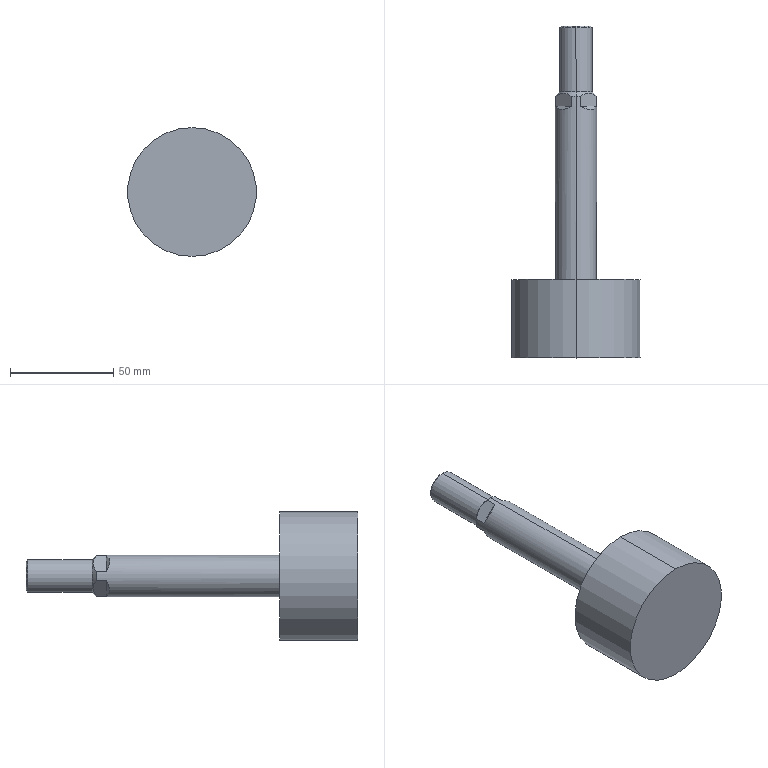Component | SolidWorks | NewCurveBenderSC63x40Cylinder-DoubleWheel-1_NewTypeCurveBenderSC-63x40(0)_r-DoubleWheel-1 | 1 solid | 21 faces | box 62.5 x 161 x 62.5 mm | volume 151202 mm3 | plane 11 | cylinder 6 | cone 4 | commonest cylinder face diameters 62.5 x2 20 x2 16 x2
build123d program:
from build123d import *

# Parameters (mm, degrees)
CUT_EXTRUDE1_DEPTH      = 17
CUT_EXTRUDE1_DEPTH_BACK = 17
CUT_EXTRUDE2_DEPTH      = 17
CUT_EXTRUDE2_DEPTH_BACK = 17


with BuildPart() as part:
    # Sketch1 → Revolve1 (revolve)
    with BuildSketch(Plane.XY, mode=Mode.PRIVATE) as revolve1_sk:
        Polygon((-57, 0), (-57, 7.08), (-56.08, 8), (-25, 8), (-23, 10), (66, 10), (66, 31.25), (104, 31.25), (104, 0), align=None)
    revolve(revolve1_sk.sketch.rotate(Axis((104, 0, 0), (-1, 0, 0)), 270), axis=Axis((104, 0, 0), (-1, 0, 0)))

    # Sketch2 → Cut-Extrude1 (cut, two sides: drawn at the far end of the back side and taken through both)
    with BuildSketch(Plane(origin=(0, 0, 0), x_dir=(1, 0, 0), z_dir=(0, -0.7071, 0.7071)).offset(-CUT_EXTRUDE1_DEPTH_BACK)):
        Polygon((-74, -25.5), (-1, -25.5), (-18, -8.5), (-57, -8.5), (-57, 8.5), (-18, 8.5), (-1, 25.5), (-74, 25.5), align=None)
    extrude(amount=CUT_EXTRUDE1_DEPTH + CUT_EXTRUDE1_DEPTH_BACK, mode=Mode.SUBTRACT)

    # Sketch3 → Cut-Extrude2 (cut, two sides: drawn at the far end of the back side and taken through both)
    with BuildSketch(Plane(origin=(0, 0, 0), x_dir=(-1, 0, 0), z_dir=(0, -0.7071, -0.7071)).offset(-CUT_EXTRUDE2_DEPTH_BACK)):
        Polygon((74, 25.5), (1, 25.5), (18, 8.5), (57, 8.5), (57, -8.5), (18, -8.5), (1, -25.5), (74, -25.5), align=None)
    extrude(amount=CUT_EXTRUDE2_DEPTH + CUT_EXTRUDE2_DEPTH_BACK, mode=Mode.SUBTRACT)


solid = part.part

# Placed as in the assembly
solid = solid.moved(Location((50, -301, 0), (0, 0, -90)))
STEP:
#1=CARTESIAN_POINT('',(1.969,-15.945,1.23));
#2=VERTEX_POINT('',#1);
#3=CARTESIAN_POINT('',(1.969,-15.945,-1.23));
#4=VERTEX_POINT('',#3);
#5=CARTESIAN_POINT('',(1.969,-15.945,0.));
#6=DIRECTION('',(-0.,1.,0.));
#7=DIRECTION('',(0.,0.,1.));
#8=AXIS2_PLACEMENT_3D('',#5,#6,#7);
#9=CIRCLE('',#8,1.23);
#10=EDGE_CURVE('',#2,#4,#9,.T.);
#11=ORIENTED_EDGE('',*,*,#10,.T.);
#12=CARTESIAN_POINT('',(1.969,-14.449,-1.23));
#13=VERTEX_POINT('',#12);
#14=CARTESIAN_POINT('',(1.969,-15.945,-1.23));
#15=DIRECTION('',(-0.,1.,0.));
#16=VECTOR('',#15,39.37);
#17=LINE('',#14,#16);
#18=EDGE_CURVE('',#4,#13,#17,.T.);
#19=ORIENTED_EDGE('',*,*,#18,.T.);
#20=CARTESIAN_POINT('',(1.969,-14.449,1.23));
#21=VERTEX_POINT('',#20);
#22=CARTESIAN_POINT('',(1.969,-14.449,0.));
#23=DIRECTION('',(-0.,1.,0.));
#24=DIRECTION('',(0.,0.,1.));
#25=AXIS2_PLACEMENT_3D('',#22,#23,#24);
#26=CIRCLE('',#25,1.23);
#27=EDGE_CURVE('',#21,#13,#26,.T.);
#28=ORIENTED_EDGE('',*,*,#27,.F.);
#29=CARTESIAN_POINT('',(1.969,-15.945,1.23));
#30=DIRECTION('',(-0.,1.,0.));
#31=VECTOR('',#30,39.37);
#32=LINE('',#29,#31);
#33=EDGE_CURVE('',#2,#21,#32,.T.);
#34=ORIENTED_EDGE('',*,*,#33,.F.);
#35=EDGE_LOOP('',(#11,#19,#28,#34));
#36=FACE_OUTER_BOUND('',#35,.T.);
#37=CARTESIAN_POINT('',(1.969,-15.945,0.));
#38=DIRECTION('',(-0.,1.,0.));
#39=DIRECTION('',(0.,0.,1.));
#40=AXIS2_PLACEMENT_3D('',#37,#38,#39);
#41=CYLINDRICAL_SURFACE('',#40,1.23);
#42=ADVANCED_FACE('',(#36),#41,.T.);
#43=CARTESIAN_POINT('',(1.969,-14.449,0.3937));
#44=VERTEX_POINT('',#43);
#45=CARTESIAN_POINT('',(1.969,-14.449,-0.3937));
#46=VERTEX_POINT('',#45);
#47=CARTESIAN_POINT('',(1.969,-14.449,0.));
#48=DIRECTION('',(-0.,1.,0.));
#49=DIRECTION('',(0.,0.,1.));
#50=AXIS2_PLACEMENT_3D('',#47,#48,#49);
#51=CIRCLE('',#50,0.3937);
#52=EDGE_CURVE('',#44,#46,#51,.T.);
#53=ORIENTED_EDGE('',*,*,#52,.T.);
#54=CARTESIAN_POINT('',(1.969,-10.945,-0.3937));
#55=VERTEX_POINT('',#54);
#56=CARTESIAN_POINT('',(1.969,-15.945,-0.3937));
#57=DIRECTION('',(-0.,1.,0.));
#58=VECTOR('',#57,39.37);
#59=LINE('',#56,#58);
#60=EDGE_CURVE('',#46,#55,#59,.T.);
#61=ORIENTED_EDGE('',*,*,#60,.T.);
#62=CARTESIAN_POINT('',(2.058,-10.945,-0.3833));
#63=VERTEX_POINT('',#62);
#64=CARTESIAN_POINT('',(1.969,-10.945,0.));
#65=DIRECTION('',(-0.,1.,0.));
#66=DIRECTION('',(0.,0.,1.));
#67=AXIS2_PLACEMENT_3D('',#64,#65,#66);
#68=CIRCLE('',#67,0.3937);
#69=EDGE_CURVE('',#63,#55,#68,.T.);
#70=ORIENTED_EDGE('',*,*,#69,.F.);
#71=CARTESIAN_POINT('',(2.058,-11.142,-0.3833));
#72=VERTEX_POINT('',#71);
#73=CARTESIAN_POINT('',(2.058,-15.945,-0.3833));
#74=DIRECTION('',(0.,-1.,-0.));
#75=VECTOR('',#74,39.37);
#76=LINE('',#73,#75);
#77=EDGE_CURVE('',#63,#72,#76,.T.);
#78=ORIENTED_EDGE('',*,*,#77,.T.);
#79=CARTESIAN_POINT('',(2.352,-11.142,-0.08998));
#80=VERTEX_POINT('',#79);
#81=CARTESIAN_POINT('',(2.058,-11.142,-0.3833));
#82=CARTESIAN_POINT('',(2.208,-11.223,-0.3482));
#83=CARTESIAN_POINT('',(2.317,-11.223,-0.2395));
#84=CARTESIAN_POINT('',(2.352,-11.142,-0.08998));
#85=(BOUNDED_CURVE()B_SPLINE_CURVE(3,(#81,#82,#83,#84),.UNSPECIFIED.,.F.,.F.)B_SPLINE_CURVE_WITH_KNOTS((4,4),(2.587,3.696),.UNSPECIFIED.)CURVE()GEOMETRIC_REPRESENTATION_ITEM()RATIONAL_B_SPLINE_CURVE((1.,0.9,0.9,1.))REPRESENTATION_ITEM(''));
#86=EDGE_CURVE('',#72,#80,#85,.T.);
#87=ORIENTED_EDGE('',*,*,#86,.T.);
#88=CARTESIAN_POINT('',(2.352,-10.945,-0.08998));
#89=VERTEX_POINT('',#88);
#90=CARTESIAN_POINT('',(2.352,-15.945,-0.08998));
#91=DIRECTION('',(-0.,1.,0.));
#92=VECTOR('',#91,39.37);
#93=LINE('',#90,#92);
#94=EDGE_CURVE('',#80,#89,#93,.T.);
#95=ORIENTED_EDGE('',*,*,#94,.T.);
#96=CARTESIAN_POINT('',(2.352,-10.945,0.08998));
#97=VERTEX_POINT('',#96);
#98=CARTESIAN_POINT('',(1.969,-10.945,0.));
#99=DIRECTION('',(-0.,1.,0.));
#100=DIRECTION('',(0.,0.,1.));
#101=AXIS2_PLACEMENT_3D('',#98,#99,#100);
#102=CIRCLE('',#101,0.3937);
#103=EDGE_CURVE('',#97,#89,#102,.T.);
#104=ORIENTED_EDGE('',*,*,#103,.F.);
#105=CARTESIAN_POINT('',(2.352,-11.142,0.08998));
#106=VERTEX_POINT('',#105);
#107=CARTESIAN_POINT('',(2.352,-15.945,0.08998));
#108=DIRECTION('',(0.,-1.,-0.));
#109=VECTOR('',#108,39.37);
#110=LINE('',#107,#109);
#111=EDGE_CURVE('',#97,#106,#110,.T.);
#112=ORIENTED_EDGE('',*,*,#111,.T.);
#113=CARTESIAN_POINT('',(2.058,-11.142,0.3833));
#114=VERTEX_POINT('',#113);
#115=CARTESIAN_POINT('',(2.352,-11.142,0.08998));
#116=CARTESIAN_POINT('',(2.317,-11.223,0.2395));
#117=CARTESIAN_POINT('',(2.208,-11.223,0.3482));
#118=CARTESIAN_POINT('',(2.058,-11.142,0.3833));
#119=(BOUNDED_CURVE()B_SPLINE_CURVE(3,(#115,#116,#117,#118),.UNSPECIFIED.,.F.,.F.)B_SPLINE_CURVE_WITH_KNOTS((4,4),(2.587,3.696),.UNSPECIFIED.)CURVE()GEOMETRIC_REPRESENTATION_ITEM()RATIONAL_B_SPLINE_CURVE((1.,0.9,0.9,1.))REPRESENTATION_ITEM(''));
#120=EDGE_CURVE('',#106,#114,#119,.T.);
#121=ORIENTED_EDGE('',*,*,#120,.T.);
#122=CARTESIAN_POINT('',(2.058,-10.945,0.3833));
#123=VERTEX_POINT('',#122);
#124=CARTESIAN_POINT('',(2.058,-15.945,0.3833));
#125=DIRECTION('',(-0.,1.,0.));
#126=VECTOR('',#125,39.37);
#127=LINE('',#124,#126);
#128=EDGE_CURVE('',#114,#123,#127,.T.);
#129=ORIENTED_EDGE('',*,*,#128,.T.);
#130=CARTESIAN_POINT('',(1.969,-10.945,0.3937));
#131=VERTEX_POINT('',#130);
#132=CARTESIAN_POINT('',(1.969,-10.945,0.));
#133=DIRECTION('',(-0.,1.,0.));
#134=DIRECTION('',(0.,0.,1.));
#135=AXIS2_PLACEMENT_3D('',#132,#133,#134);
#136=CIRCLE('',#135,0.3937);
#137=EDGE_CURVE('',#131,#123,#136,.T.);
#138=ORIENTED_EDGE('',*,*,#137,.F.);
#139=CARTESIAN_POINT('',(1.969,-15.945,0.3937));
#140=DIRECTION('',(-0.,1.,0.));
#141=VECTOR('',#140,39.37);
#142=LINE('',#139,#141);
#143=EDGE_CURVE('',#44,#131,#142,.T.);
#144=ORIENTED_EDGE('',*,*,#143,.F.);
#145=EDGE_LOOP('',(#53,#61,#70,#78,#87,#95,#104,#112,#121,#129,#138,#144));
#146=FACE_OUTER_BOUND('',#145,.T.);
#147=CARTESIAN_POINT('',(1.969,-15.945,0.));
#148=DIRECTION('',(-0.,1.,0.));
#149=DIRECTION('',(0.,0.,1.));
#150=AXIS2_PLACEMENT_3D('',#147,#148,#149);
#151=CYLINDRICAL_SURFACE('',#150,0.3937);
#152=ADVANCED_FACE('',(#146),#151,.T.);
#153=CARTESIAN_POINT('',(1.969,-10.866,0.315));
#154=VERTEX_POINT('',#153);
#155=CARTESIAN_POINT('',(1.969,-10.866,-0.315));
#156=VERTEX_POINT('',#155);
#157=CARTESIAN_POINT('',(1.969,-10.866,0.));
#158=DIRECTION('',(-0.,1.,0.));
#159=DIRECTION('',(0.,0.,1.));
#160=AXIS2_PLACEMENT_3D('',#157,#158,#159);
#161=CIRCLE('',#160,0.315);
#162=EDGE_CURVE('',#154,#156,#161,.T.);
#163=ORIENTED_EDGE('',*,*,#162,.F.);
#164=CARTESIAN_POINT('',(1.969,-10.945,0.3937));
#165=DIRECTION('',(0.,-0.7071,0.7071));
#166=VECTOR('',#165,39.37);
#167=LINE('',#164,#166);
#168=EDGE_CURVE('',#154,#131,#167,.T.);
#169=ORIENTED_EDGE('',*,*,#168,.T.);
#170=ORIENTED_EDGE('',*,*,#137,.T.);
#171=CARTESIAN_POINT('',(2.058,-10.945,0.3833));
#172=CARTESIAN_POINT('',(2.081,-10.928,0.3605));
#173=CARTESIAN_POINT('',(2.105,-10.913,0.337));
#174=CARTESIAN_POINT('',(2.141,-10.897,0.3003));
#175=CARTESIAN_POINT('',(2.154,-10.893,0.2878));
#176=CARTESIAN_POINT('',(2.18,-10.887,0.2622));
#177=CARTESIAN_POINT('',(2.192,-10.886,0.2494));
#178=CARTESIAN_POINT('',(2.218,-10.886,0.2239));
#179=CARTESIAN_POINT('',(2.231,-10.887,0.2111));
#180=CARTESIAN_POINT('',(2.256,-10.893,0.1855));
#181=CARTESIAN_POINT('',(2.269,-10.897,0.173));
#182=CARTESIAN_POINT('',(2.306,-10.913,0.1362));
#183=CARTESIAN_POINT('',(2.329,-10.928,0.1128));
#184=CARTESIAN_POINT('',(2.352,-10.945,0.08998));
#185=B_SPLINE_CURVE_WITH_KNOTS('',3,(#171,#172,#173,#174,#175,#176,#177,#178,#179,#180,#181,#182,#183,#184),.UNSPECIFIED.,.F.,.F.,(4,2,2,2,2,2,4),(0.00000043,0.002754,0.004131,0.005507,0.006884,0.008261,0.01101),.UNSPECIFIED.);
#186=EDGE_CURVE('',#123,#97,#185,.T.);
#187=ORIENTED_EDGE('',*,*,#186,.T.);
#188=ORIENTED_EDGE('',*,*,#103,.T.);
#189=CARTESIAN_POINT('',(2.352,-10.945,-0.08998));
#190=CARTESIAN_POINT('',(2.329,-10.928,-0.1128));
#191=CARTESIAN_POINT('',(2.306,-10.913,-0.1362));
#192=CARTESIAN_POINT('',(2.269,-10.897,-0.1729));
#193=CARTESIAN_POINT('',(2.256,-10.893,-0.1855));
#194=CARTESIAN_POINT('',(2.231,-10.887,-0.211));
#195=CARTESIAN_POINT('',(2.218,-10.886,-0.2238));
#196=CARTESIAN_POINT('',(2.192,-10.886,-0.2494));
#197=CARTESIAN_POINT('',(2.18,-10.887,-0.2622));
#198=CARTESIAN_POINT('',(2.154,-10.893,-0.2877));
#199=CARTESIAN_POINT('',(2.141,-10.897,-0.3003));
#200=CARTESIAN_POINT('',(2.105,-10.913,-0.337));
#201=CARTESIAN_POINT('',(2.081,-10.928,-0.3605));
#202=CARTESIAN_POINT('',(2.058,-10.945,-0.3833));
#203=B_SPLINE_CURVE_WITH_KNOTS('',3,(#189,#190,#191,#192,#193,#194,#195,#196,#197,#198,#199,#200,#201,#202),.UNSPECIFIED.,.F.,.F.,(4,2,2,2,2,2,4),(0.00000043,0.002754,0.004131,0.005507,0.006884,0.008261,0.01101),.UNSPECIFIED.);
#204=EDGE_CURVE('',#89,#63,#203,.T.);
#205=ORIENTED_EDGE('',*,*,#204,.T.);
#206=ORIENTED_EDGE('',*,*,#69,.T.);
#207=CARTESIAN_POINT('',(1.969,-10.945,-0.3937));
#208=DIRECTION('',(0.,-0.7071,-0.7071));
#209=VECTOR('',#208,39.37);
#210=LINE('',#207,#209);
#211=EDGE_CURVE('',#156,#55,#210,.T.);
#212=ORIENTED_EDGE('',*,*,#211,.F.);
#213=EDGE_LOOP('',(#163,#169,#170,#187,#188,#205,#206,#212));
#214=FACE_OUTER_BOUND('',#213,.T.);
#215=CARTESIAN_POINT('',(1.969,-10.945,0.));
#216=DIRECTION('',(0.,-1.,-0.));
#217=DIRECTION('',(0.,0.,-1.));
#218=AXIS2_PLACEMENT_3D('',#215,#216,#217);
#219=CONICAL_SURFACE('',#218,0.3937,0.7854);
#220=ADVANCED_FACE('',(#214),#219,.T.);
#221=ORIENTED_EDGE('',*,*,#162,.T.);
#222=CARTESIAN_POINT('',(1.969,-9.643,-0.315));
#223=VERTEX_POINT('',#222);
#224=CARTESIAN_POINT('',(1.969,-15.945,-0.315));
#225=DIRECTION('',(-0.,1.,0.));
#226=VECTOR('',#225,39.37);
#227=LINE('',#224,#226);
#228=EDGE_CURVE('',#156,#223,#227,.T.);
#229=ORIENTED_EDGE('',*,*,#228,.T.);
#230=CARTESIAN_POINT('',(1.969,-9.643,0.315));
#231=VERTEX_POINT('',#230);
#232=CARTESIAN_POINT('',(1.969,-9.643,0.));
#233=DIRECTION('',(-0.,1.,0.));
#234=DIRECTION('',(0.,0.,1.));
#235=AXIS2_PLACEMENT_3D('',#232,#233,#234);
#236=CIRCLE('',#235,0.315);
#237=EDGE_CURVE('',#231,#223,#236,.T.);
#238=ORIENTED_EDGE('',*,*,#237,.F.);
#239=CARTESIAN_POINT('',(1.969,-15.945,0.315));
#240=DIRECTION('',(-0.,1.,0.));
#241=VECTOR('',#240,39.37);
#242=LINE('',#239,#241);
#243=EDGE_CURVE('',#154,#231,#242,.T.);
#244=ORIENTED_EDGE('',*,*,#243,.F.);
#245=EDGE_LOOP('',(#221,#229,#238,#244));
#246=FACE_OUTER_BOUND('',#245,.T.);
#247=CARTESIAN_POINT('',(1.969,-15.945,0.));
#248=DIRECTION('',(-0.,1.,0.));
#249=DIRECTION('',(0.,0.,1.));
#250=AXIS2_PLACEMENT_3D('',#247,#248,#249);
#251=CYLINDRICAL_SURFACE('',#250,0.315);
#252=ADVANCED_FACE('',(#246),#251,.T.);
#253=CARTESIAN_POINT('',(1.969,-9.606,0.2787));
#254=VERTEX_POINT('',#253);
#255=CARTESIAN_POINT('',(1.969,-9.606,-0.2787));
#256=VERTEX_POINT('',#255);
#257=CARTESIAN_POINT('',(1.969,-9.606,0.));
#258=DIRECTION('',(-0.,1.,0.));
#259=DIRECTION('',(0.,0.,1.));
#260=AXIS2_PLACEMENT_3D('',#257,#258,#259);
#261=CIRCLE('',#260,0.2787);
#262=EDGE_CURVE('',#254,#256,#261,.T.);
#263=ORIENTED_EDGE('',*,*,#262,.F.);
#264=CARTESIAN_POINT('',(1.969,-9.643,0.315));
#265=DIRECTION('',(0.,-0.7071,0.7071));
#266=VECTOR('',#265,39.37);
#267=LINE('',#264,#266);
#268=EDGE_CURVE('',#254,#231,#267,.T.);
#269=ORIENTED_EDGE('',*,*,#268,.T.);
#270=ORIENTED_EDGE('',*,*,#237,.T.);
#271=CARTESIAN_POINT('',(1.969,-9.643,-0.315));
#272=DIRECTION('',(0.,-0.7071,-0.7071));
#273=VECTOR('',#272,39.37);
#274=LINE('',#271,#273);
#275=EDGE_CURVE('',#256,#223,#274,.T.);
#276=ORIENTED_EDGE('',*,*,#275,.F.);
#277=EDGE_LOOP('',(#263,#269,#270,#276));
#278=FACE_OUTER_BOUND('',#277,.T.);
#279=CARTESIAN_POINT('',(1.969,-9.643,0.));
#280=DIRECTION('',(0.,-1.,-0.));
#281=DIRECTION('',(0.,0.,-1.));
#282=AXIS2_PLACEMENT_3D('',#279,#280,#281);
#283=CONICAL_SURFACE('',#282,0.315,0.7854);
#284=ADVANCED_FACE('',(#278),#283,.T.);
#285=CARTESIAN_POINT('',(1.969,-9.606,0.));
#286=DIRECTION('',(-0.,1.,0.));
#287=DIRECTION('',(0.,0.,1.));
#288=AXIS2_PLACEMENT_3D('',#285,#286,#287);
#289=CIRCLE('',#288,0.2787);
#290=EDGE_CURVE('',#256,#254,#289,.T.);
#291=ORIENTED_EDGE('',*,*,#290,.T.);
#292=ORIENTED_EDGE('',*,*,#262,.T.);
#293=EDGE_LOOP('',(#291,#292));
#294=FACE_OUTER_BOUND('',#293,.T.);
#295=CARTESIAN_POINT('',(1.969,-9.606,0.));
#296=DIRECTION('',(0.,-1.,0.));
#297=DIRECTION('',(0.,-0.,-1.));
#298=AXIS2_PLACEMENT_3D('',#295,#296,#297);
#299=PLANE('',#298);
#300=ADVANCED_FACE('',(#294),#299,.F.);
#301=ORIENTED_EDGE('',*,*,#268,.F.);
#302=ORIENTED_EDGE('',*,*,#290,.F.);
#303=ORIENTED_EDGE('',*,*,#275,.T.);
#304=CARTESIAN_POINT('',(1.969,-9.643,0.));
#305=DIRECTION('',(-0.,1.,0.));
#306=DIRECTION('',(0.,0.,1.));
#307=AXIS2_PLACEMENT_3D('',#304,#305,#306);
#308=CIRCLE('',#307,0.315);
#309=EDGE_CURVE('',#223,#231,#308,.T.);
#310=ORIENTED_EDGE('',*,*,#309,.T.);
#311=EDGE_LOOP('',(#301,#302,#303,#310));
#312=FACE_OUTER_BOUND('',#311,.T.);
#313=CARTESIAN_POINT('',(1.969,-9.643,0.));
#314=DIRECTION('',(0.,-1.,-0.));
#315=DIRECTION('',(0.,0.,-1.));
#316=AXIS2_PLACEMENT_3D('',#313,#314,#315);
#317=CONICAL_SURFACE('',#316,0.315,0.7854);
#318=ADVANCED_FACE('',(#312),#317,.T.);
#319=ORIENTED_EDGE('',*,*,#228,.F.);
#320=CARTESIAN_POINT('',(1.969,-10.866,0.));
#321=DIRECTION('',(-0.,1.,0.));
#322=DIRECTION('',(0.,0.,1.));
#323=AXIS2_PLACEMENT_3D('',#320,#321,#322);
#324=CIRCLE('',#323,0.315);
#325=EDGE_CURVE('',#156,#154,#324,.T.);
#326=ORIENTED_EDGE('',*,*,#325,.T.);
#327=ORIENTED_EDGE('',*,*,#243,.T.);
#328=ORIENTED_EDGE('',*,*,#309,.F.);
#329=EDGE_LOOP('',(#319,#326,#327,#328));
#330=FACE_OUTER_BOUND('',#329,.T.);
#331=CARTESIAN_POINT('',(1.969,-15.945,0.));
#332=DIRECTION('',(-0.,1.,0.));
#333=DIRECTION('',(0.,0.,1.));
#334=AXIS2_PLACEMENT_3D('',#331,#332,#333);
#335=CYLINDRICAL_SURFACE('',#334,0.315);
#336=ADVANCED_FACE('',(#330),#335,.T.);
#337=ORIENTED_EDGE('',*,*,#168,.F.);
#338=ORIENTED_EDGE('',*,*,#325,.F.);
#339=ORIENTED_EDGE('',*,*,#211,.T.);
#340=CARTESIAN_POINT('',(1.879,-10.945,-0.3833));
#341=VERTEX_POINT('',#340);
#342=CARTESIAN_POINT('',(1.969,-10.945,0.));
#343=DIRECTION('',(-0.,1.,0.));
#344=DIRECTION('',(0.,0.,1.));
#345=AXIS2_PLACEMENT_3D('',#342,#343,#344);
#346=CIRCLE('',#345,0.3937);
#347=EDGE_CURVE('',#55,#341,#346,.T.);
#348=ORIENTED_EDGE('',*,*,#347,.T.);
#349=CARTESIAN_POINT('',(1.585,-10.945,-0.08998));
#350=VERTEX_POINT('',#349);
#351=CARTESIAN_POINT('',(1.879,-10.945,-0.3833));
#352=CARTESIAN_POINT('',(1.856,-10.928,-0.3605));
#353=CARTESIAN_POINT('',(1.832,-10.913,-0.337));
#354=CARTESIAN_POINT('',(1.796,-10.897,-0.3003));
#355=CARTESIAN_POINT('',(1.783,-10.893,-0.2878));
#356=CARTESIAN_POINT('',(1.757,-10.887,-0.2622));
#357=CARTESIAN_POINT('',(1.745,-10.886,-0.2494));
#358=CARTESIAN_POINT('',(1.719,-10.886,-0.2239));
#359=CARTESIAN_POINT('',(1.706,-10.887,-0.2111));
#360=CARTESIAN_POINT('',(1.681,-10.893,-0.1855));
#361=CARTESIAN_POINT('',(1.668,-10.897,-0.173));
#362=CARTESIAN_POINT('',(1.631,-10.913,-0.1362));
#363=CARTESIAN_POINT('',(1.608,-10.928,-0.1128));
#364=CARTESIAN_POINT('',(1.585,-10.945,-0.08998));
#365=B_SPLINE_CURVE_WITH_KNOTS('',3,(#351,#352,#353,#354,#355,#356,#357,#358,#359,#360,#361,#362,#363,#364),.UNSPECIFIED.,.F.,.F.,(4,2,2,2,2,2,4),(0.00000043,0.002754,0.004131,0.005507,0.006884,0.008261,0.01101),.UNSPECIFIED.);
#366=EDGE_CURVE('',#341,#350,#365,.T.);
#367=ORIENTED_EDGE('',*,*,#366,.T.);
#368=CARTESIAN_POINT('',(1.585,-10.945,0.08998));
#369=VERTEX_POINT('',#368);
#370=CARTESIAN_POINT('',(1.969,-10.945,0.));
#371=DIRECTION('',(-0.,1.,0.));
#372=DIRECTION('',(0.,0.,1.));
#373=AXIS2_PLACEMENT_3D('',#370,#371,#372);
#374=CIRCLE('',#373,0.3937);
#375=EDGE_CURVE('',#350,#369,#374,.T.);
#376=ORIENTED_EDGE('',*,*,#375,.T.);
#377=CARTESIAN_POINT('',(1.879,-10.945,0.3833));
#378=VERTEX_POINT('',#377);
#379=CARTESIAN_POINT('',(1.585,-10.945,0.08998));
#380=CARTESIAN_POINT('',(1.608,-10.928,0.1128));
#381=CARTESIAN_POINT('',(1.631,-10.913,0.1362));
#382=CARTESIAN_POINT('',(1.668,-10.897,0.1729));
#383=CARTESIAN_POINT('',(1.681,-10.893,0.1855));
#384=CARTESIAN_POINT('',(1.706,-10.887,0.211));
#385=CARTESIAN_POINT('',(1.719,-10.886,0.2238));
#386=CARTESIAN_POINT('',(1.745,-10.886,0.2494));
#387=CARTESIAN_POINT('',(1.757,-10.887,0.2622));
#388=CARTESIAN_POINT('',(1.783,-10.893,0.2877));
#389=CARTESIAN_POINT('',(1.796,-10.897,0.3003));
#390=CARTESIAN_POINT('',(1.832,-10.913,0.337));
#391=CARTESIAN_POINT('',(1.856,-10.928,0.3605));
#392=CARTESIAN_POINT('',(1.879,-10.945,0.3833));
#393=B_SPLINE_CURVE_WITH_KNOTS('',3,(#379,#380,#381,#382,#383,#384,#385,#386,#387,#388,#389,#390,#391,#392),.UNSPECIFIED.,.F.,.F.,(4,2,2,2,2,2,4),(0.00000043,0.002754,0.004131,0.005507,0.006884,0.008261,0.01101),.UNSPECIFIED.);
#394=EDGE_CURVE('',#369,#378,#393,.T.);
#395=ORIENTED_EDGE('',*,*,#394,.T.);
#396=CARTESIAN_POINT('',(1.969,-10.945,0.));
#397=DIRECTION('',(-0.,1.,0.));
#398=DIRECTION('',(0.,0.,1.));
#399=AXIS2_PLACEMENT_3D('',#396,#397,#398);
#400=CIRCLE('',#399,0.3937);
#401=EDGE_CURVE('',#378,#131,#400,.T.);
#402=ORIENTED_EDGE('',*,*,#401,.T.);
#403=EDGE_LOOP('',(#337,#338,#339,#348,#367,#376,#395,#402));
#404=FACE_OUTER_BOUND('',#403,.T.);
#405=CARTESIAN_POINT('',(1.969,-10.945,0.));
#406=DIRECTION('',(0.,-1.,-0.));
#407=DIRECTION('',(0.,0.,-1.));
#408=AXIS2_PLACEMENT_3D('',#405,#406,#407);
#409=CONICAL_SURFACE('',#408,0.3937,0.7854);
#410=ADVANCED_FACE('',(#404),#409,.T.);
#411=ORIENTED_EDGE('',*,*,#60,.F.);
#412=CARTESIAN_POINT('',(1.969,-14.449,0.));
#413=DIRECTION('',(-0.,1.,0.));
#414=DIRECTION('',(0.,0.,1.));
#415=AXIS2_PLACEMENT_3D('',#412,#413,#414);
#416=CIRCLE('',#415,0.3937);
#417=EDGE_CURVE('',#46,#44,#416,.T.);
#418=ORIENTED_EDGE('',*,*,#417,.T.);
#419=ORIENTED_EDGE('',*,*,#143,.T.);
#420=ORIENTED_EDGE('',*,*,#401,.F.);
#421=CARTESIAN_POINT('',(1.879,-11.142,0.3833));
#422=VERTEX_POINT('',#421);
#423=CARTESIAN_POINT('',(1.879,-15.945,0.3833));
#424=DIRECTION('',(0.,-1.,-0.));
#425=VECTOR('',#424,39.37);
#426=LINE('',#423,#425);
#427=EDGE_CURVE('',#378,#422,#426,.T.);
#428=ORIENTED_EDGE('',*,*,#427,.T.);
#429=CARTESIAN_POINT('',(1.585,-11.142,0.08998));
#430=VERTEX_POINT('',#429);
#431=CARTESIAN_POINT('',(1.879,-11.142,0.3833));
#432=CARTESIAN_POINT('',(1.729,-11.223,0.3482));
#433=CARTESIAN_POINT('',(1.62,-11.223,0.2395));
#434=CARTESIAN_POINT('',(1.585,-11.142,0.08998));
#435=(BOUNDED_CURVE()B_SPLINE_CURVE(3,(#431,#432,#433,#434),.UNSPECIFIED.,.F.,.F.)B_SPLINE_CURVE_WITH_KNOTS((4,4),(2.587,3.696),.UNSPECIFIED.)CURVE()GEOMETRIC_REPRESENTATION_ITEM()RATIONAL_B_SPLINE_CURVE((1.,0.9,0.9,1.))REPRESENTATION_ITEM(''));
#436=EDGE_CURVE('',#422,#430,#435,.T.);
#437=ORIENTED_EDGE('',*,*,#436,.T.);
#438=CARTESIAN_POINT('',(1.585,-15.945,0.08998));
#439=DIRECTION('',(-0.,1.,0.));
#440=VECTOR('',#439,39.37);
#441=LINE('',#438,#440);
#442=EDGE_CURVE('',#430,#369,#441,.T.);
#443=ORIENTED_EDGE('',*,*,#442,.T.);
#444=ORIENTED_EDGE('',*,*,#375,.F.);
#445=CARTESIAN_POINT('',(1.585,-11.142,-0.08998));
#446=VERTEX_POINT('',#445);
#447=CARTESIAN_POINT('',(1.585,-15.945,-0.08998));
#448=DIRECTION('',(0.,-1.,-0.));
#449=VECTOR('',#448,39.37);
#450=LINE('',#447,#449);
#451=EDGE_CURVE('',#350,#446,#450,.T.);
#452=ORIENTED_EDGE('',*,*,#451,.T.);
#453=CARTESIAN_POINT('',(1.879,-11.142,-0.3833));
#454=VERTEX_POINT('',#453);
#455=CARTESIAN_POINT('',(1.585,-11.142,-0.08998));
#456=CARTESIAN_POINT('',(1.62,-11.223,-0.2395));
#457=CARTESIAN_POINT('',(1.729,-11.223,-0.3482));
#458=CARTESIAN_POINT('',(1.879,-11.142,-0.3833));
#459=(BOUNDED_CURVE()B_SPLINE_CURVE(3,(#455,#456,#457,#458),.UNSPECIFIED.,.F.,.T.)B_SPLINE_CURVE_WITH_KNOTS((4,4),(2.587,3.696),.UNSPECIFIED.)CURVE()GEOMETRIC_REPRESENTATION_ITEM()RATIONAL_B_SPLINE_CURVE((1.,0.9,0.9,1.))REPRESENTATION_ITEM(''));
#460=EDGE_CURVE('',#446,#454,#459,.T.);
#461=ORIENTED_EDGE('',*,*,#460,.T.);
#462=CARTESIAN_POINT('',(1.879,-15.945,-0.3833));
#463=DIRECTION('',(-0.,1.,0.));
#464=VECTOR('',#463,39.37);
#465=LINE('',#462,#464);
#466=EDGE_CURVE('',#454,#341,#465,.T.);
#467=ORIENTED_EDGE('',*,*,#466,.T.);
#468=ORIENTED_EDGE('',*,*,#347,.F.);
#469=EDGE_LOOP('',(#411,#418,#419,#420,#428,#437,#443,#444,#452,#461,#467,#468));
#470=FACE_OUTER_BOUND('',#469,.T.);
#471=CARTESIAN_POINT('',(1.969,-15.945,0.));
#472=DIRECTION('',(-0.,1.,0.));
#473=DIRECTION('',(0.,0.,1.));
#474=AXIS2_PLACEMENT_3D('',#471,#472,#473);
#475=CYLINDRICAL_SURFACE('',#474,0.3937);
#476=ADVANCED_FACE('',(#470),#475,.T.);
#477=ORIENTED_EDGE('',*,*,#52,.F.);
#478=ORIENTED_EDGE('',*,*,#417,.F.);
#479=EDGE_LOOP('',(#477,#478));
#480=FACE_BOUND('',#479,.T.);
#481=ORIENTED_EDGE('',*,*,#27,.T.);
#482=CARTESIAN_POINT('',(1.969,-14.449,0.));
#483=DIRECTION('',(-0.,1.,0.));
#484=DIRECTION('',(0.,0.,1.));
#485=AXIS2_PLACEMENT_3D('',#482,#483,#484);
#486=CIRCLE('',#485,1.23);
#487=EDGE_CURVE('',#13,#21,#486,.T.);
#488=ORIENTED_EDGE('',*,*,#487,.T.);
#489=EDGE_LOOP('',(#481,#488));
#490=FACE_OUTER_BOUND('',#489,.T.);
#491=CARTESIAN_POINT('',(2.362,-14.449,0.));
#492=DIRECTION('',(0.,-1.,0.));
#493=DIRECTION('',(0.,-0.,-1.));
#494=AXIS2_PLACEMENT_3D('',#491,#492,#493);
#495=PLANE('',#494);
#496=ADVANCED_FACE('',(#480,#490),#495,.F.);
#497=ORIENTED_EDGE('',*,*,#18,.F.);
#498=CARTESIAN_POINT('',(1.969,-15.945,0.));
#499=DIRECTION('',(-0.,1.,0.));
#500=DIRECTION('',(0.,0.,1.));
#501=AXIS2_PLACEMENT_3D('',#498,#499,#500);
#502=CIRCLE('',#501,1.23);
#503=EDGE_CURVE('',#4,#2,#502,.T.);
#504=ORIENTED_EDGE('',*,*,#503,.T.);
#505=ORIENTED_EDGE('',*,*,#33,.T.);
#506=ORIENTED_EDGE('',*,*,#487,.F.);
#507=EDGE_LOOP('',(#497,#504,#505,#506));
#508=FACE_OUTER_BOUND('',#507,.T.);
#509=CARTESIAN_POINT('',(1.969,-15.945,0.));
#510=DIRECTION('',(-0.,1.,0.));
#511=DIRECTION('',(0.,0.,1.));
#512=AXIS2_PLACEMENT_3D('',#509,#510,#511);
#513=CYLINDRICAL_SURFACE('',#512,1.23);
#514=ADVANCED_FACE('',(#508),#513,.T.);
#515=ORIENTED_EDGE('',*,*,#10,.F.);
#516=ORIENTED_EDGE('',*,*,#503,.F.);
#517=EDGE_LOOP('',(#515,#516));
#518=FACE_OUTER_BOUND('',#517,.T.);
#519=CARTESIAN_POINT('',(3.199,-15.945,0.));
#520=DIRECTION('',(-0.,1.,-0.));
#521=DIRECTION('',(0.,0.,1.));
#522=AXIS2_PLACEMENT_3D('',#519,#520,#521);
#523=PLANE('',#522);
#524=ADVANCED_FACE('',(#518),#523,.F.);
#525=CARTESIAN_POINT('',(2.205,-11.142,-0.7099));
#526=DIRECTION('',(-0.7071,-0.,0.7071));
#527=VECTOR('',#526,39.37);
#528=LINE('',#525,#527);
#529=EDGE_CURVE('',#454,#446,#528,.T.);
#530=ORIENTED_EDGE('',*,*,#529,.F.);
#531=ORIENTED_EDGE('',*,*,#460,.F.);
#532=EDGE_LOOP('',(#530,#531));
#533=FACE_OUTER_BOUND('',#532,.T.);
#534=CARTESIAN_POINT('',(1.732,-11.811,-1.183));
#535=DIRECTION('',(0.5,-0.7071,0.5));
#536=DIRECTION('',(0.,-0.5774,-0.8165));
#537=AXIS2_PLACEMENT_3D('',#534,#535,#536);
#538=PLANE('',#537);
#539=ADVANCED_FACE('',(#533),#538,.F.);
#540=ORIENTED_EDGE('',*,*,#529,.T.);
#541=ORIENTED_EDGE('',*,*,#451,.F.);
#542=ORIENTED_EDGE('',*,*,#366,.F.);
#543=ORIENTED_EDGE('',*,*,#466,.F.);
#544=EDGE_LOOP('',(#540,#541,#542,#543));
#545=FACE_OUTER_BOUND('',#544,.T.);
#546=CARTESIAN_POINT('',(2.205,-11.142,-0.7099));
#547=DIRECTION('',(0.7071,0.,0.7071));
#548=DIRECTION('',(-0.7071,-0.,0.7071));
#549=AXIS2_PLACEMENT_3D('',#546,#547,#548);
#550=PLANE('',#549);
#551=ADVANCED_FACE('',(#545),#550,.F.);
#552=CARTESIAN_POINT('',(2.678,-11.142,-0.2366));
#553=DIRECTION('',(-0.7071,-0.,0.7071));
#554=VECTOR('',#553,39.37);
#555=LINE('',#552,#554);
#556=EDGE_CURVE('',#106,#114,#555,.T.);
#557=ORIENTED_EDGE('',*,*,#556,.T.);
#558=ORIENTED_EDGE('',*,*,#120,.F.);
#559=EDGE_LOOP('',(#557,#558));
#560=FACE_OUTER_BOUND('',#559,.T.);
#561=CARTESIAN_POINT('',(2.678,-11.142,-0.2366));
#562=DIRECTION('',(-0.5,-0.7071,-0.5));
#563=DIRECTION('',(-0.,0.5774,-0.8165));
#564=AXIS2_PLACEMENT_3D('',#561,#562,#563);
#565=PLANE('',#564);
#566=ADVANCED_FACE('',(#560),#565,.F.);
#567=ORIENTED_EDGE('',*,*,#556,.F.);
#568=ORIENTED_EDGE('',*,*,#111,.F.);
#569=ORIENTED_EDGE('',*,*,#186,.F.);
#570=ORIENTED_EDGE('',*,*,#128,.F.);
#571=EDGE_LOOP('',(#567,#568,#569,#570));
#572=FACE_OUTER_BOUND('',#571,.T.);
#573=CARTESIAN_POINT('',(2.678,-9.606,-0.2366));
#574=DIRECTION('',(-0.7071,-0.,-0.7071));
#575=DIRECTION('',(0.7071,0.,-0.7071));
#576=AXIS2_PLACEMENT_3D('',#573,#574,#575);
#577=PLANE('',#576);
#578=ADVANCED_FACE('',(#572),#577,.F.);
#579=CARTESIAN_POINT('',(2.678,-11.142,0.2366));
#580=DIRECTION('',(-0.7071,-0.,-0.7071));
#581=VECTOR('',#580,39.37);
#582=LINE('',#579,#581);
#583=EDGE_CURVE('',#80,#72,#582,.T.);
#584=ORIENTED_EDGE('',*,*,#583,.F.);
#585=ORIENTED_EDGE('',*,*,#86,.F.);
#586=EDGE_LOOP('',(#584,#585));
#587=FACE_OUTER_BOUND('',#586,.T.);
#588=CARTESIAN_POINT('',(3.152,-11.811,-0.2366));
#589=DIRECTION('',(-0.5,-0.7071,0.5));
#590=DIRECTION('',(0.,-0.5774,-0.8165));
#591=AXIS2_PLACEMENT_3D('',#588,#589,#590);
#592=PLANE('',#591);
#593=ADVANCED_FACE('',(#587),#592,.F.);
#594=ORIENTED_EDGE('',*,*,#583,.T.);
#595=ORIENTED_EDGE('',*,*,#77,.F.);
#596=ORIENTED_EDGE('',*,*,#204,.F.);
#597=ORIENTED_EDGE('',*,*,#94,.F.);
#598=EDGE_LOOP('',(#594,#595,#596,#597));
#599=FACE_OUTER_BOUND('',#598,.T.);
#600=CARTESIAN_POINT('',(2.678,-11.142,0.2366));
#601=DIRECTION('',(-0.7071,-0.,0.7071));
#602=DIRECTION('',(-0.7071,-0.,-0.7071));
#603=AXIS2_PLACEMENT_3D('',#600,#601,#602);
#604=PLANE('',#603);
#605=ADVANCED_FACE('',(#599),#604,.F.);
#606=CARTESIAN_POINT('',(2.205,-11.142,0.7099));
#607=DIRECTION('',(-0.7071,-0.,-0.7071));
#608=VECTOR('',#607,39.37);
#609=LINE('',#606,#608);
#610=EDGE_CURVE('',#422,#430,#609,.T.);
#611=ORIENTED_EDGE('',*,*,#610,.T.);
#612=ORIENTED_EDGE('',*,*,#436,.F.);
#613=EDGE_LOOP('',(#611,#612));
#614=FACE_OUTER_BOUND('',#613,.T.);
#615=CARTESIAN_POINT('',(2.205,-11.142,0.7099));
#616=DIRECTION('',(0.5,-0.7071,-0.5));
#617=DIRECTION('',(-0.,0.5774,-0.8165));
#618=AXIS2_PLACEMENT_3D('',#615,#616,#617);
#619=PLANE('',#618);
#620=ADVANCED_FACE('',(#614),#619,.F.);
#621=ORIENTED_EDGE('',*,*,#610,.F.);
#622=ORIENTED_EDGE('',*,*,#427,.F.);
#623=ORIENTED_EDGE('',*,*,#394,.F.);
#624=ORIENTED_EDGE('',*,*,#442,.F.);
#625=EDGE_LOOP('',(#621,#622,#623,#624));
#626=FACE_OUTER_BOUND('',#625,.T.);
#627=CARTESIAN_POINT('',(2.205,-9.606,0.7099));
#628=DIRECTION('',(0.7071,0.,-0.7071));
#629=DIRECTION('',(0.7071,0.,0.7071));
#630=AXIS2_PLACEMENT_3D('',#627,#628,#629);
#631=PLANE('',#630);
#632=ADVANCED_FACE('',(#626),#631,.F.);
#633=CLOSED_SHELL('',(#42,#152,#220,#252,#284,#300,#318,#336,#410,#476,#496,#514,#524,#539,#551,#566,#578,#593,#605,#620,#632));
#634=MANIFOLD_SOLID_BREP('',#633);
#635=CARTESIAN_POINT('',(0.,0.,0.));
#636=DIRECTION('',(0.,0.,1.));
#637=DIRECTION('',(1.,0.,0.));
#638=AXIS2_PLACEMENT_3D('',#635,#636,#637);
#639=(LENGTH_UNIT()NAMED_UNIT(*)SI_UNIT($,.METRE.));
#640=LENGTH_MEASURE_WITH_UNIT(LENGTH_MEASURE(0.0254),#639);
#641=DIMENSIONAL_EXPONENTS(1.,0.,0.,0.,0.,0.,0.);
#642=(CONVERSION_BASED_UNIT('',#640)LENGTH_UNIT()NAMED_UNIT(#641));
#643=UNCERTAINTY_MEASURE_WITH_UNIT(LENGTH_MEASURE(0.00001),#642,'','');
#644=(NAMED_UNIT(*)PLANE_ANGLE_UNIT()SI_UNIT($,.RADIAN.));
#645=(NAMED_UNIT(*)SI_UNIT($,.STERADIAN.)SOLID_ANGLE_UNIT());
#646=(GEOMETRIC_REPRESENTATION_CONTEXT(3)GLOBAL_UNCERTAINTY_ASSIGNED_CONTEXT((#643))GLOBAL_UNIT_ASSIGNED_CONTEXT((#642,#644,#645))REPRESENTATION_CONTEXT('',''));
#647=ADVANCED_BREP_SHAPE_REPRESENTATION('',(#634,#638),#646);
#648=COLOUR_RGB('',0.7922,0.8196,0.9333);
#649=FILL_AREA_STYLE_COLOUR('',#648);
#650=FILL_AREA_STYLE('',(#649));
#651=SURFACE_STYLE_FILL_AREA(#650);
#652=SURFACE_SIDE_STYLE('',(#651));
#653=SURFACE_STYLE_USAGE(.BOTH.,#652);
#654=PRESENTATION_STYLE_ASSIGNMENT((#653));
#655=STYLED_ITEM('',(#654),#634);
#656=(LENGTH_UNIT()NAMED_UNIT(*)SI_UNIT($,.METRE.));
#657=LENGTH_MEASURE_WITH_UNIT(LENGTH_MEASURE(0.0254),#656);
#658=DIMENSIONAL_EXPONENTS(1.,0.,0.,0.,0.,0.,0.);
#659=(CONVERSION_BASED_UNIT('',#657)LENGTH_UNIT()NAMED_UNIT(#658));
#660=UNCERTAINTY_MEASURE_WITH_UNIT(LENGTH_MEASURE(0.00001),#659,'','');
#661=(NAMED_UNIT(*)PLANE_ANGLE_UNIT()SI_UNIT($,.RADIAN.));
#662=(NAMED_UNIT(*)SI_UNIT($,.STERADIAN.)SOLID_ANGLE_UNIT());
#663=(GEOMETRIC_REPRESENTATION_CONTEXT(3)GLOBAL_UNCERTAINTY_ASSIGNED_CONTEXT((#660))GLOBAL_UNIT_ASSIGNED_CONTEXT((#659,#661,#662))REPRESENTATION_CONTEXT('',''));
#664=MECHANICAL_DESIGN_GEOMETRIC_PRESENTATION_REPRESENTATION('',(#655),#663);
#665=PRESENTATION_LAYER_ASSIGNMENT('','',(#655));